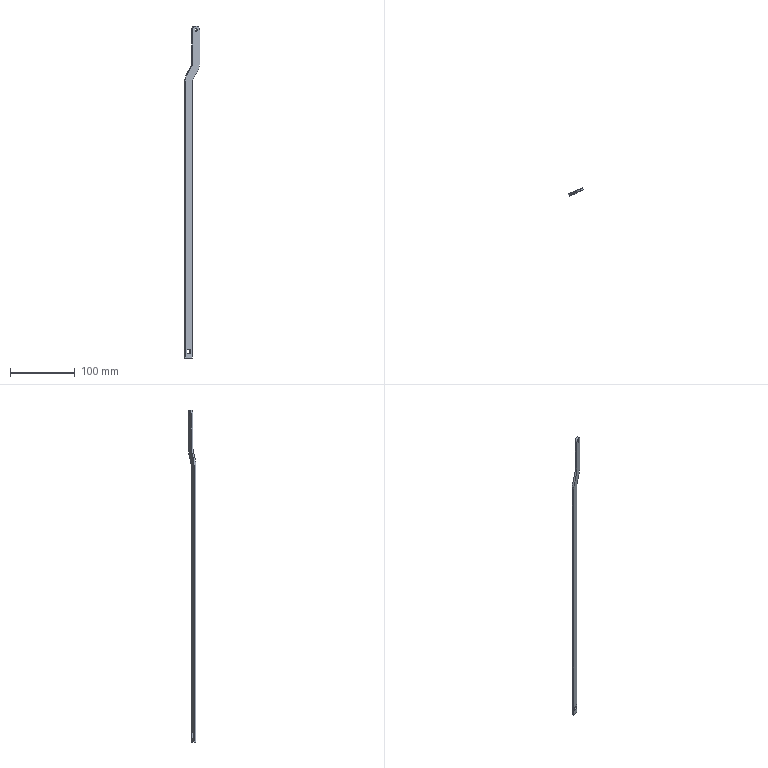Component | SolidWorks | RightDoorAssembly-1_LinkRodLock-1_UpperLinkRod-1 | 1 solid | 21 faces | box 23.38 x 11.77 x 511 mm | volume 18287 mm3 | plane 13 | cylinder 8 | commonest cylinder face diameters 4.2 x2 12 x2 10 x2 34 x2
STEP:
#1=COLOUR_RGB('',0.7922,0.8196,0.9333);
#2=FILL_AREA_STYLE_COLOUR('',#1);
#3=FILL_AREA_STYLE('',(#2));
#4=SURFACE_STYLE_FILL_AREA(#3);
#5=SURFACE_SIDE_STYLE('',(#4));
#6=SURFACE_STYLE_USAGE(.BOTH.,#5);
#7=PRESENTATION_STYLE_ASSIGNMENT((#6));
#8=CARTESIAN_POINT('',(-12.373,15.98,59.984));
#9=VERTEX_POINT('',#8);
#10=CARTESIAN_POINT('',(-12.373,15.98,60.15));
#11=VERTEX_POINT('',#10);
#12=CARTESIAN_POINT('',(-12.373,15.98,60.067));
#13=DIRECTION('',(-0.3744,0.9273,-0.));
#14=DIRECTION('',(0.,0.,1.));
#15=AXIS2_PLACEMENT_3D('',#12,#13,#14);
#16=CIRCLE('',#15,0.08268);
#17=EDGE_CURVE('',#9,#11,#16,.T.);
#18=ORIENTED_EDGE('',*,*,#17,.F.);
#19=CARTESIAN_POINT('',(-12.417,16.09,59.984));
#20=VERTEX_POINT('',#19);
#21=CARTESIAN_POINT('',(-12.373,15.98,59.984));
#22=DIRECTION('',(-0.3744,0.9273,-0.));
#23=VECTOR('',#22,39.37);
#24=LINE('',#21,#23);
#25=EDGE_CURVE('',#9,#20,#24,.T.);
#26=ORIENTED_EDGE('',*,*,#25,.T.);
#27=CARTESIAN_POINT('',(-12.417,16.09,60.15));
#28=VERTEX_POINT('',#27);
#29=CARTESIAN_POINT('',(-12.417,16.09,60.067));
#30=DIRECTION('',(-0.3744,0.9273,-0.));
#31=DIRECTION('',(0.,0.,1.));
#32=AXIS2_PLACEMENT_3D('',#29,#30,#31);
#33=CIRCLE('',#32,0.08268);
#34=EDGE_CURVE('',#20,#28,#33,.T.);
#35=ORIENTED_EDGE('',*,*,#34,.T.);
#36=CARTESIAN_POINT('',(-12.373,15.98,60.15));
#37=DIRECTION('',(-0.3744,0.9273,-0.));
#38=VECTOR('',#37,39.37);
#39=LINE('',#36,#38);
#40=EDGE_CURVE('',#11,#28,#39,.T.);
#41=ORIENTED_EDGE('',*,*,#40,.F.);
#42=EDGE_LOOP('',(#18,#26,#35,#41));
#43=FACE_OUTER_BOUND('',#42,.T.);
#44=CARTESIAN_POINT('',(-12.373,15.98,60.067));
#45=DIRECTION('',(-0.3744,0.9273,-0.));
#46=DIRECTION('',(0.,0.,1.));
#47=AXIS2_PLACEMENT_3D('',#44,#45,#46);
#48=CYLINDRICAL_SURFACE('',#47,0.08268);
#49=ADVANCED_FACE('',(#43),#48,.F.);
#50=CARTESIAN_POINT('',(-12.592,15.892,60.067));
#51=VERTEX_POINT('',#50);
#52=CARTESIAN_POINT('',(-12.373,15.98,60.303));
#53=VERTEX_POINT('',#52);
#54=CARTESIAN_POINT('',(-12.373,15.98,60.067));
#55=DIRECTION('',(-0.3744,0.9273,-0.));
#56=DIRECTION('',(-0.,0.,1.));
#57=AXIS2_PLACEMENT_3D('',#54,#55,#56);
#58=CIRCLE('',#57,0.2362);
#59=EDGE_CURVE('',#51,#53,#58,.T.);
#60=ORIENTED_EDGE('',*,*,#59,.T.);
#61=CARTESIAN_POINT('',(-12.417,16.09,60.303));
#62=VERTEX_POINT('',#61);
#63=CARTESIAN_POINT('',(-12.373,15.98,60.303));
#64=DIRECTION('',(-0.3744,0.9273,-0.));
#65=VECTOR('',#64,39.37);
#66=LINE('',#63,#65);
#67=EDGE_CURVE('',#53,#62,#66,.T.);
#68=ORIENTED_EDGE('',*,*,#67,.T.);
#69=CARTESIAN_POINT('',(-12.636,16.001,60.067));
#70=VERTEX_POINT('',#69);
#71=CARTESIAN_POINT('',(-12.417,16.09,60.067));
#72=DIRECTION('',(-0.3744,0.9273,-0.));
#73=DIRECTION('',(-0.,0.,1.));
#74=AXIS2_PLACEMENT_3D('',#71,#72,#73);
#75=CIRCLE('',#74,0.2362);
#76=EDGE_CURVE('',#70,#62,#75,.T.);
#77=ORIENTED_EDGE('',*,*,#76,.F.);
#78=CARTESIAN_POINT('',(-12.592,15.892,60.067));
#79=DIRECTION('',(-0.3744,0.9273,-0.));
#80=VECTOR('',#79,39.37);
#81=LINE('',#78,#80);
#82=EDGE_CURVE('',#51,#70,#81,.T.);
#83=ORIENTED_EDGE('',*,*,#82,.F.);
#84=EDGE_LOOP('',(#60,#68,#77,#83));
#85=FACE_OUTER_BOUND('',#84,.T.);
#86=CARTESIAN_POINT('',(-12.373,15.98,60.067));
#87=DIRECTION('',(-0.3744,0.9273,-0.));
#88=DIRECTION('',(-0.,0.,1.));
#89=AXIS2_PLACEMENT_3D('',#86,#87,#88);
#90=CYLINDRICAL_SURFACE('',#89,0.2362);
#91=ADVANCED_FACE('',(#85),#90,.T.);
#92=CARTESIAN_POINT('',(-13.074,15.824,40.185));
#93=VERTEX_POINT('',#92);
#94=CARTESIAN_POINT('',(-13.074,15.824,56.942));
#95=VERTEX_POINT('',#94);
#96=CARTESIAN_POINT('',(-13.074,15.824,40.185));
#97=DIRECTION('',(-0.,0.,1.));
#98=VECTOR('',#97,39.37);
#99=LINE('',#96,#98);
#100=EDGE_CURVE('',#93,#95,#99,.T.);
#101=ORIENTED_EDGE('',*,*,#100,.F.);
#102=CARTESIAN_POINT('',(-13.03,15.715,40.185));
#103=VERTEX_POINT('',#102);
#104=CARTESIAN_POINT('',(-13.03,15.715,40.185));
#105=DIRECTION('',(-0.3744,0.9273,-0.));
#106=VECTOR('',#105,39.37);
#107=LINE('',#104,#106);
#108=EDGE_CURVE('',#103,#93,#107,.T.);
#109=ORIENTED_EDGE('',*,*,#108,.F.);
#110=CARTESIAN_POINT('',(-13.03,15.715,56.942));
#111=VERTEX_POINT('',#110);
#112=CARTESIAN_POINT('',(-13.03,15.715,40.185));
#113=DIRECTION('',(-0.,0.,1.));
#114=VECTOR('',#113,39.37);
#115=LINE('',#112,#114);
#116=EDGE_CURVE('',#103,#111,#115,.T.);
#117=ORIENTED_EDGE('',*,*,#116,.T.);
#118=CARTESIAN_POINT('',(-13.03,15.715,56.942));
#119=DIRECTION('',(-0.3744,0.9273,-0.));
#120=VECTOR('',#119,39.37);
#121=LINE('',#118,#120);
#122=EDGE_CURVE('',#111,#95,#121,.T.);
#123=ORIENTED_EDGE('',*,*,#122,.T.);
#124=EDGE_LOOP('',(#101,#109,#117,#123));
#125=FACE_OUTER_BOUND('',#124,.T.);
#126=CARTESIAN_POINT('',(-13.03,15.715,40.185));
#127=DIRECTION('',(-0.9273,-0.3744,-0.));
#128=DIRECTION('',(-0.,0.,1.));
#129=AXIS2_PLACEMENT_3D('',#126,#127,#128);
#130=PLANE('',#129);
#131=ADVANCED_FACE('',(#125),#130,.T.);
#132=CARTESIAN_POINT('',(-12.636,16.001,40.185));
#133=VERTEX_POINT('',#132);
#134=CARTESIAN_POINT('',(-12.636,16.001,40.185));
#135=DIRECTION('',(-0.9273,-0.3744,-0.));
#136=VECTOR('',#135,39.37);
#137=LINE('',#134,#136);
#138=EDGE_CURVE('',#133,#93,#137,.T.);
#139=ORIENTED_EDGE('',*,*,#138,.F.);
#140=CARTESIAN_POINT('',(-12.592,15.892,40.185));
#141=VERTEX_POINT('',#140);
#142=CARTESIAN_POINT('',(-12.592,15.892,40.185));
#143=DIRECTION('',(-0.3744,0.9273,-0.));
#144=VECTOR('',#143,39.37);
#145=LINE('',#142,#144);
#146=EDGE_CURVE('',#141,#133,#145,.T.);
#147=ORIENTED_EDGE('',*,*,#146,.F.);
#148=CARTESIAN_POINT('',(-12.592,15.892,40.185));
#149=DIRECTION('',(-0.9273,-0.3744,-0.));
#150=VECTOR('',#149,39.37);
#151=LINE('',#148,#150);
#152=EDGE_CURVE('',#141,#103,#151,.T.);
#153=ORIENTED_EDGE('',*,*,#152,.T.);
#154=ORIENTED_EDGE('',*,*,#108,.T.);
#155=EDGE_LOOP('',(#139,#147,#153,#154));
#156=FACE_OUTER_BOUND('',#155,.T.);
#157=CARTESIAN_POINT('',(-12.592,15.892,40.185));
#158=DIRECTION('',(0.,-0.,-1.));
#159=DIRECTION('',(-0.3744,0.9273,-0.));
#160=AXIS2_PLACEMENT_3D('',#157,#158,#159);
#161=PLANE('',#160);
#162=ADVANCED_FACE('',(#156),#161,.T.);
#163=CARTESIAN_POINT('',(-12.636,16.001,56.942));
#164=VERTEX_POINT('',#163);
#165=CARTESIAN_POINT('',(-12.636,16.001,40.185));
#166=DIRECTION('',(0.,-0.,-1.));
#167=VECTOR('',#166,39.37);
#168=LINE('',#165,#167);
#169=EDGE_CURVE('',#164,#133,#168,.T.);
#170=ORIENTED_EDGE('',*,*,#169,.F.);
#171=CARTESIAN_POINT('',(-12.592,15.892,56.942));
#172=VERTEX_POINT('',#171);
#173=CARTESIAN_POINT('',(-12.592,15.892,56.942));
#174=DIRECTION('',(-0.3744,0.9273,-0.));
#175=VECTOR('',#174,39.37);
#176=LINE('',#173,#175);
#177=EDGE_CURVE('',#172,#164,#176,.T.);
#178=ORIENTED_EDGE('',*,*,#177,.F.);
#179=CARTESIAN_POINT('',(-12.592,15.892,40.185));
#180=DIRECTION('',(0.,-0.,-1.));
#181=VECTOR('',#180,39.37);
#182=LINE('',#179,#181);
#183=EDGE_CURVE('',#172,#141,#182,.T.);
#184=ORIENTED_EDGE('',*,*,#183,.T.);
#185=ORIENTED_EDGE('',*,*,#146,.T.);
#186=EDGE_LOOP('',(#170,#178,#184,#185));
#187=FACE_OUTER_BOUND('',#186,.T.);
#188=CARTESIAN_POINT('',(-12.592,15.892,40.185));
#189=DIRECTION('',(0.9273,0.3744,0.));
#190=DIRECTION('',(0.,-0.,-1.));
#191=AXIS2_PLACEMENT_3D('',#188,#189,#190);
#192=PLANE('',#191);
#193=ADVANCED_FACE('',(#187),#192,.T.);
#194=CARTESIAN_POINT('',(-12.612,16.011,57.04));
#195=VERTEX_POINT('',#194);
#196=CARTESIAN_POINT('',(-12.454,16.075,56.942));
#197=DIRECTION('',(0.3744,-0.9273,0.));
#198=DIRECTION('',(-0.,0.,1.));
#199=AXIS2_PLACEMENT_3D('',#196,#197,#198);
#200=CIRCLE('',#199,0.1969);
#201=EDGE_CURVE('',#195,#164,#200,.T.);
#202=ORIENTED_EDGE('',*,*,#201,.F.);
#203=CARTESIAN_POINT('',(-12.568,15.902,57.04));
#204=VERTEX_POINT('',#203);
#205=CARTESIAN_POINT('',(-12.568,15.902,57.04));
#206=DIRECTION('',(-0.3744,0.9273,-0.));
#207=VECTOR('',#206,39.37);
#208=LINE('',#205,#207);
#209=EDGE_CURVE('',#204,#195,#208,.T.);
#210=ORIENTED_EDGE('',*,*,#209,.F.);
#211=CARTESIAN_POINT('',(-12.41,15.965,56.942));
#212=DIRECTION('',(0.3744,-0.9273,0.));
#213=DIRECTION('',(-0.,0.,1.));
#214=AXIS2_PLACEMENT_3D('',#211,#212,#213);
#215=CIRCLE('',#214,0.1969);
#216=EDGE_CURVE('',#204,#172,#215,.T.);
#217=ORIENTED_EDGE('',*,*,#216,.T.);
#218=ORIENTED_EDGE('',*,*,#177,.T.);
#219=EDGE_LOOP('',(#202,#210,#217,#218));
#220=FACE_OUTER_BOUND('',#219,.T.);
#221=CARTESIAN_POINT('',(-12.41,15.965,56.942));
#222=DIRECTION('',(-0.3744,0.9273,-0.));
#223=DIRECTION('',(-0.,0.,1.));
#224=AXIS2_PLACEMENT_3D('',#221,#222,#223);
#225=CYLINDRICAL_SURFACE('',#224,0.1969);
#226=ADVANCED_FACE('',(#220),#225,.F.);
#227=CARTESIAN_POINT('',(-12.281,16.145,57.657));
#228=VERTEX_POINT('',#227);
#229=CARTESIAN_POINT('',(-12.281,16.145,57.657));
#230=DIRECTION('',(-0.4636,-0.1872,-0.866));
#231=VECTOR('',#230,39.37);
#232=LINE('',#229,#231);
#233=EDGE_CURVE('',#228,#195,#232,.T.);
#234=ORIENTED_EDGE('',*,*,#233,.F.);
#235=CARTESIAN_POINT('',(-12.237,16.035,57.657));
#236=VERTEX_POINT('',#235);
#237=CARTESIAN_POINT('',(-12.237,16.035,57.657));
#238=DIRECTION('',(-0.3744,0.9273,-0.));
#239=VECTOR('',#238,39.37);
#240=LINE('',#237,#239);
#241=EDGE_CURVE('',#236,#228,#240,.T.);
#242=ORIENTED_EDGE('',*,*,#241,.F.);
#243=CARTESIAN_POINT('',(-12.237,16.035,57.657));
#244=DIRECTION('',(-0.4636,-0.1872,-0.866));
#245=VECTOR('',#244,39.37);
#246=LINE('',#243,#245);
#247=EDGE_CURVE('',#236,#204,#246,.T.);
#248=ORIENTED_EDGE('',*,*,#247,.T.);
#249=ORIENTED_EDGE('',*,*,#209,.T.);
#250=EDGE_LOOP('',(#234,#242,#248,#249));
#251=FACE_OUTER_BOUND('',#250,.T.);
#252=CARTESIAN_POINT('',(-12.237,16.035,57.657));
#253=DIRECTION('',(0.803,0.3242,-0.5));
#254=DIRECTION('',(-0.4636,-0.1872,-0.866));
#255=AXIS2_PLACEMENT_3D('',#252,#253,#254);
#256=PLANE('',#255);
#257=ADVANCED_FACE('',(#251),#256,.T.);
#258=CARTESIAN_POINT('',(-12.198,16.178,57.992));
#259=VERTEX_POINT('',#258);
#260=CARTESIAN_POINT('',(-12.819,15.928,57.992));
#261=DIRECTION('',(-0.3744,0.9273,-0.));
#262=DIRECTION('',(-0.,0.,1.));
#263=AXIS2_PLACEMENT_3D('',#260,#261,#262);
#264=CIRCLE('',#263,0.6693);
#265=EDGE_CURVE('',#259,#228,#264,.T.);
#266=ORIENTED_EDGE('',*,*,#265,.F.);
#267=CARTESIAN_POINT('',(-12.154,16.069,57.992));
#268=VERTEX_POINT('',#267);
#269=CARTESIAN_POINT('',(-12.154,16.069,57.992));
#270=DIRECTION('',(-0.3744,0.9273,-0.));
#271=VECTOR('',#270,39.37);
#272=LINE('',#269,#271);
#273=EDGE_CURVE('',#268,#259,#272,.T.);
#274=ORIENTED_EDGE('',*,*,#273,.F.);
#275=CARTESIAN_POINT('',(-12.775,15.818,57.992));
#276=DIRECTION('',(-0.3744,0.9273,-0.));
#277=DIRECTION('',(-0.,0.,1.));
#278=AXIS2_PLACEMENT_3D('',#275,#276,#277);
#279=CIRCLE('',#278,0.6693);
#280=EDGE_CURVE('',#268,#236,#279,.T.);
#281=ORIENTED_EDGE('',*,*,#280,.T.);
#282=ORIENTED_EDGE('',*,*,#241,.T.);
#283=EDGE_LOOP('',(#266,#274,#281,#282));
#284=FACE_OUTER_BOUND('',#283,.T.);
#285=CARTESIAN_POINT('',(-12.775,15.818,57.992));
#286=DIRECTION('',(-0.3744,0.9273,-0.));
#287=DIRECTION('',(-0.,0.,1.));
#288=AXIS2_PLACEMENT_3D('',#285,#286,#287);
#289=CYLINDRICAL_SURFACE('',#288,0.6693);
#290=ADVANCED_FACE('',(#284),#289,.T.);
#291=CARTESIAN_POINT('',(-12.198,16.178,60.067));
#292=VERTEX_POINT('',#291);
#293=CARTESIAN_POINT('',(-12.198,16.178,57.992));
#294=DIRECTION('',(0.,-0.,-1.));
#295=VECTOR('',#294,39.37);
#296=LINE('',#293,#295);
#297=EDGE_CURVE('',#292,#259,#296,.T.);
#298=ORIENTED_EDGE('',*,*,#297,.F.);
#299=CARTESIAN_POINT('',(-12.154,16.069,60.067));
#300=VERTEX_POINT('',#299);
#301=CARTESIAN_POINT('',(-12.154,16.069,60.067));
#302=DIRECTION('',(-0.3744,0.9273,-0.));
#303=VECTOR('',#302,39.37);
#304=LINE('',#301,#303);
#305=EDGE_CURVE('',#300,#292,#304,.T.);
#306=ORIENTED_EDGE('',*,*,#305,.F.);
#307=CARTESIAN_POINT('',(-12.154,16.069,57.992));
#308=DIRECTION('',(0.,-0.,-1.));
#309=VECTOR('',#308,39.37);
#310=LINE('',#307,#309);
#311=EDGE_CURVE('',#300,#268,#310,.T.);
#312=ORIENTED_EDGE('',*,*,#311,.T.);
#313=ORIENTED_EDGE('',*,*,#273,.T.);
#314=EDGE_LOOP('',(#298,#306,#312,#313));
#315=FACE_OUTER_BOUND('',#314,.T.);
#316=CARTESIAN_POINT('',(-12.154,16.069,57.992));
#317=DIRECTION('',(0.9273,0.3744,0.));
#318=DIRECTION('',(0.,-0.,-1.));
#319=AXIS2_PLACEMENT_3D('',#316,#317,#318);
#320=PLANE('',#319);
#321=ADVANCED_FACE('',(#315),#320,.T.);
#322=ORIENTED_EDGE('',*,*,#67,.F.);
#323=CARTESIAN_POINT('',(-12.373,15.98,60.067));
#324=DIRECTION('',(-0.3744,0.9273,-0.));
#325=DIRECTION('',(-0.,0.,1.));
#326=AXIS2_PLACEMENT_3D('',#323,#324,#325);
#327=CIRCLE('',#326,0.2362);
#328=EDGE_CURVE('',#53,#300,#327,.T.);
#329=ORIENTED_EDGE('',*,*,#328,.T.);
#330=ORIENTED_EDGE('',*,*,#305,.T.);
#331=CARTESIAN_POINT('',(-12.417,16.09,60.067));
#332=DIRECTION('',(-0.3744,0.9273,-0.));
#333=DIRECTION('',(-0.,0.,1.));
#334=AXIS2_PLACEMENT_3D('',#331,#332,#333);
#335=CIRCLE('',#334,0.2362);
#336=EDGE_CURVE('',#62,#292,#335,.T.);
#337=ORIENTED_EDGE('',*,*,#336,.F.);
#338=EDGE_LOOP('',(#322,#329,#330,#337));
#339=FACE_OUTER_BOUND('',#338,.T.);
#340=CARTESIAN_POINT('',(-12.373,15.98,60.067));
#341=DIRECTION('',(-0.3744,0.9273,-0.));
#342=DIRECTION('',(-0.,0.,1.));
#343=AXIS2_PLACEMENT_3D('',#340,#341,#342);
#344=CYLINDRICAL_SURFACE('',#343,0.2362);
#345=ADVANCED_FACE('',(#339),#344,.T.);
#346=CARTESIAN_POINT('',(-12.636,16.001,57.992));
#347=VERTEX_POINT('',#346);
#348=CARTESIAN_POINT('',(-12.636,16.001,57.992));
#349=DIRECTION('',(0.,0.,1.));
#350=VECTOR('',#349,39.37);
#351=LINE('',#348,#350);
#352=EDGE_CURVE('',#347,#70,#351,.T.);
#353=ORIENTED_EDGE('',*,*,#352,.F.);
#354=CARTESIAN_POINT('',(-12.592,15.892,57.992));
#355=VERTEX_POINT('',#354);
#356=CARTESIAN_POINT('',(-12.592,15.892,57.992));
#357=DIRECTION('',(-0.3744,0.9273,-0.));
#358=VECTOR('',#357,39.37);
#359=LINE('',#356,#358);
#360=EDGE_CURVE('',#355,#347,#359,.T.);
#361=ORIENTED_EDGE('',*,*,#360,.F.);
#362=CARTESIAN_POINT('',(-12.592,15.892,57.992));
#363=DIRECTION('',(0.,0.,1.));
#364=VECTOR('',#363,39.37);
#365=LINE('',#362,#364);
#366=EDGE_CURVE('',#355,#51,#365,.T.);
#367=ORIENTED_EDGE('',*,*,#366,.T.);
#368=ORIENTED_EDGE('',*,*,#82,.T.);
#369=EDGE_LOOP('',(#353,#361,#367,#368));
#370=FACE_OUTER_BOUND('',#369,.T.);
#371=CARTESIAN_POINT('',(-12.592,15.892,57.992));
#372=DIRECTION('',(-0.9273,-0.3744,0.));
#373=DIRECTION('',(0.,0.,1.));
#374=AXIS2_PLACEMENT_3D('',#371,#372,#373);
#375=PLANE('',#374);
#376=ADVANCED_FACE('',(#370),#375,.T.);
#377=CARTESIAN_POINT('',(-12.661,15.991,57.894));
#378=VERTEX_POINT('',#377);
#379=CARTESIAN_POINT('',(-12.819,15.928,57.992));
#380=DIRECTION('',(0.3744,-0.9273,0.));
#381=DIRECTION('',(-0.,0.,1.));
#382=AXIS2_PLACEMENT_3D('',#379,#380,#381);
#383=CIRCLE('',#382,0.1969);
#384=EDGE_CURVE('',#378,#347,#383,.T.);
#385=ORIENTED_EDGE('',*,*,#384,.F.);
#386=CARTESIAN_POINT('',(-12.617,15.882,57.894));
#387=VERTEX_POINT('',#386);
#388=CARTESIAN_POINT('',(-12.617,15.882,57.894));
#389=DIRECTION('',(-0.3744,0.9273,-0.));
#390=VECTOR('',#389,39.37);
#391=LINE('',#388,#390);
#392=EDGE_CURVE('',#387,#378,#391,.T.);
#393=ORIENTED_EDGE('',*,*,#392,.F.);
#394=CARTESIAN_POINT('',(-12.775,15.818,57.992));
#395=DIRECTION('',(0.3744,-0.9273,0.));
#396=DIRECTION('',(-0.,0.,1.));
#397=AXIS2_PLACEMENT_3D('',#394,#395,#396);
#398=CIRCLE('',#397,0.1969);
#399=EDGE_CURVE('',#387,#355,#398,.T.);
#400=ORIENTED_EDGE('',*,*,#399,.T.);
#401=ORIENTED_EDGE('',*,*,#360,.T.);
#402=EDGE_LOOP('',(#385,#393,#400,#401));
#403=FACE_OUTER_BOUND('',#402,.T.);
#404=CARTESIAN_POINT('',(-12.775,15.818,57.992));
#405=DIRECTION('',(-0.3744,0.9273,-0.));
#406=DIRECTION('',(-0.,0.,1.));
#407=AXIS2_PLACEMENT_3D('',#404,#405,#406);
#408=CYLINDRICAL_SURFACE('',#407,0.1969);
#409=ADVANCED_FACE('',(#403),#408,.F.);
#410=CARTESIAN_POINT('',(-12.991,15.858,57.276));
#411=VERTEX_POINT('',#410);
#412=CARTESIAN_POINT('',(-12.661,15.991,57.894));
#413=DIRECTION('',(0.4636,0.1872,0.866));
#414=VECTOR('',#413,39.37);
#415=LINE('',#412,#414);
#416=EDGE_CURVE('',#411,#378,#415,.T.);
#417=ORIENTED_EDGE('',*,*,#416,.F.);
#418=CARTESIAN_POINT('',(-12.947,15.748,57.276));
#419=VERTEX_POINT('',#418);
#420=CARTESIAN_POINT('',(-12.947,15.748,57.276));
#421=DIRECTION('',(-0.3744,0.9273,-0.));
#422=VECTOR('',#421,39.37);
#423=LINE('',#420,#422);
#424=EDGE_CURVE('',#419,#411,#423,.T.);
#425=ORIENTED_EDGE('',*,*,#424,.F.);
#426=CARTESIAN_POINT('',(-12.617,15.882,57.894));
#427=DIRECTION('',(0.4636,0.1872,0.866));
#428=VECTOR('',#427,39.37);
#429=LINE('',#426,#428);
#430=EDGE_CURVE('',#419,#387,#429,.T.);
#431=ORIENTED_EDGE('',*,*,#430,.T.);
#432=ORIENTED_EDGE('',*,*,#392,.T.);
#433=EDGE_LOOP('',(#417,#425,#431,#432));
#434=FACE_OUTER_BOUND('',#433,.T.);
#435=CARTESIAN_POINT('',(-12.617,15.882,57.894));
#436=DIRECTION('',(-0.803,-0.3242,0.5));
#437=DIRECTION('',(0.4636,0.1872,0.866));
#438=AXIS2_PLACEMENT_3D('',#435,#436,#437);
#439=PLANE('',#438);
#440=ADVANCED_FACE('',(#434),#439,.T.);
#441=CARTESIAN_POINT('',(-12.454,16.075,56.942));
#442=DIRECTION('',(-0.3744,0.9273,-0.));
#443=DIRECTION('',(-0.,0.,1.));
#444=AXIS2_PLACEMENT_3D('',#441,#442,#443);
#445=CIRCLE('',#444,0.6693);
#446=EDGE_CURVE('',#95,#411,#445,.T.);
#447=ORIENTED_EDGE('',*,*,#446,.F.);
#448=ORIENTED_EDGE('',*,*,#122,.F.);
#449=CARTESIAN_POINT('',(-12.41,15.965,56.942));
#450=DIRECTION('',(-0.3744,0.9273,-0.));
#451=DIRECTION('',(-0.,0.,1.));
#452=AXIS2_PLACEMENT_3D('',#449,#450,#451);
#453=CIRCLE('',#452,0.6693);
#454=EDGE_CURVE('',#111,#419,#453,.T.);
#455=ORIENTED_EDGE('',*,*,#454,.T.);
#456=ORIENTED_EDGE('',*,*,#424,.T.);
#457=EDGE_LOOP('',(#447,#448,#455,#456));
#458=FACE_OUTER_BOUND('',#457,.T.);
#459=CARTESIAN_POINT('',(-12.41,15.965,56.942));
#460=DIRECTION('',(-0.3744,0.9273,-0.));
#461=DIRECTION('',(-0.,0.,1.));
#462=AXIS2_PLACEMENT_3D('',#459,#460,#461);
#463=CYLINDRICAL_SURFACE('',#462,0.6693);
#464=ADVANCED_FACE('',(#458),#463,.T.);
#465=CARTESIAN_POINT('',(-12.373,15.98,60.067));
#466=DIRECTION('',(-0.3744,0.9273,-0.));
#467=DIRECTION('',(0.,0.,1.));
#468=AXIS2_PLACEMENT_3D('',#465,#466,#467);
#469=CIRCLE('',#468,0.08268);
#470=EDGE_CURVE('',#11,#9,#469,.T.);
#471=ORIENTED_EDGE('',*,*,#470,.T.);
#472=ORIENTED_EDGE('',*,*,#17,.T.);
#473=EDGE_LOOP('',(#471,#472));
#474=FACE_BOUND('',#473,.T.);
#475=CARTESIAN_POINT('',(-12.93,15.755,40.707));
#476=VERTEX_POINT('',#475);
#477=CARTESIAN_POINT('',(-12.693,15.851,40.707));
#478=VERTEX_POINT('',#477);
#479=CARTESIAN_POINT('',(-12.693,15.851,40.707));
#480=DIRECTION('',(0.9273,0.3744,0.));
#481=VECTOR('',#480,39.37);
#482=LINE('',#479,#481);
#483=EDGE_CURVE('',#476,#478,#482,.T.);
#484=ORIENTED_EDGE('',*,*,#483,.T.);
#485=CARTESIAN_POINT('',(-12.693,15.851,40.451));
#486=VERTEX_POINT('',#485);
#487=CARTESIAN_POINT('',(-12.693,15.851,40.451));
#488=DIRECTION('',(0.,-0.,-1.));
#489=VECTOR('',#488,39.37);
#490=LINE('',#487,#489);
#491=EDGE_CURVE('',#478,#486,#490,.T.);
#492=ORIENTED_EDGE('',*,*,#491,.T.);
#493=CARTESIAN_POINT('',(-12.93,15.755,40.451));
#494=VERTEX_POINT('',#493);
#495=CARTESIAN_POINT('',(-12.93,15.755,40.451));
#496=DIRECTION('',(-0.9273,-0.3744,-0.));
#497=VECTOR('',#496,39.37);
#498=LINE('',#495,#497);
#499=EDGE_CURVE('',#486,#494,#498,.T.);
#500=ORIENTED_EDGE('',*,*,#499,.T.);
#501=CARTESIAN_POINT('',(-12.93,15.755,40.707));
#502=DIRECTION('',(-0.,0.,1.));
#503=VECTOR('',#502,39.37);
#504=LINE('',#501,#503);
#505=EDGE_CURVE('',#494,#476,#504,.T.);
#506=ORIENTED_EDGE('',*,*,#505,.T.);
#507=EDGE_LOOP('',(#484,#492,#500,#506));
#508=FACE_BOUND('',#507,.T.);
#509=ORIENTED_EDGE('',*,*,#116,.F.);
#510=ORIENTED_EDGE('',*,*,#152,.F.);
#511=ORIENTED_EDGE('',*,*,#183,.F.);
#512=ORIENTED_EDGE('',*,*,#216,.F.);
#513=ORIENTED_EDGE('',*,*,#247,.F.);
#514=ORIENTED_EDGE('',*,*,#280,.F.);
#515=ORIENTED_EDGE('',*,*,#311,.F.);
#516=ORIENTED_EDGE('',*,*,#328,.F.);
#517=ORIENTED_EDGE('',*,*,#59,.F.);
#518=ORIENTED_EDGE('',*,*,#366,.F.);
#519=ORIENTED_EDGE('',*,*,#399,.F.);
#520=ORIENTED_EDGE('',*,*,#430,.F.);
#521=ORIENTED_EDGE('',*,*,#454,.F.);
#522=EDGE_LOOP('',(#509,#510,#511,#512,#513,#514,#515,#516,#517,#518,#519,#520,#521));
#523=FACE_OUTER_BOUND('',#522,.T.);
#524=CARTESIAN_POINT('',(-12.41,15.965,56.942));
#525=DIRECTION('',(-0.3744,0.9273,-0.));
#526=DIRECTION('',(-0.,0.,1.));
#527=AXIS2_PLACEMENT_3D('',#524,#525,#526);
#528=PLANE('',#527);
#529=ADVANCED_FACE('',(#474,#508,#523),#528,.F.);
#530=CARTESIAN_POINT('',(-12.417,16.09,60.067));
#531=DIRECTION('',(-0.3744,0.9273,-0.));
#532=DIRECTION('',(0.,0.,1.));
#533=AXIS2_PLACEMENT_3D('',#530,#531,#532);
#534=CIRCLE('',#533,0.08268);
#535=EDGE_CURVE('',#28,#20,#534,.T.);
#536=ORIENTED_EDGE('',*,*,#535,.F.);
#537=ORIENTED_EDGE('',*,*,#34,.F.);
#538=EDGE_LOOP('',(#536,#537));
#539=FACE_BOUND('',#538,.T.);
#540=CARTESIAN_POINT('',(-12.737,15.961,40.707));
#541=VERTEX_POINT('',#540);
#542=CARTESIAN_POINT('',(-12.737,15.961,40.451));
#543=VERTEX_POINT('',#542);
#544=CARTESIAN_POINT('',(-12.737,15.961,40.451));
#545=DIRECTION('',(0.,-0.,-1.));
#546=VECTOR('',#545,39.37);
#547=LINE('',#544,#546);
#548=EDGE_CURVE('',#541,#543,#547,.T.);
#549=ORIENTED_EDGE('',*,*,#548,.F.);
#550=CARTESIAN_POINT('',(-12.974,15.865,40.707));
#551=VERTEX_POINT('',#550);
#552=CARTESIAN_POINT('',(-12.737,15.961,40.707));
#553=DIRECTION('',(0.9273,0.3744,0.));
#554=VECTOR('',#553,39.37);
#555=LINE('',#552,#554);
#556=EDGE_CURVE('',#551,#541,#555,.T.);
#557=ORIENTED_EDGE('',*,*,#556,.F.);
#558=CARTESIAN_POINT('',(-12.974,15.865,40.451));
#559=VERTEX_POINT('',#558);
#560=CARTESIAN_POINT('',(-12.974,15.865,40.707));
#561=DIRECTION('',(-0.,0.,1.));
#562=VECTOR('',#561,39.37);
#563=LINE('',#560,#562);
#564=EDGE_CURVE('',#559,#551,#563,.T.);
#565=ORIENTED_EDGE('',*,*,#564,.F.);
#566=CARTESIAN_POINT('',(-12.974,15.865,40.451));
#567=DIRECTION('',(-0.9273,-0.3744,-0.));
#568=VECTOR('',#567,39.37);
#569=LINE('',#566,#568);
#570=EDGE_CURVE('',#543,#559,#569,.T.);
#571=ORIENTED_EDGE('',*,*,#570,.F.);
#572=EDGE_LOOP('',(#549,#557,#565,#571));
#573=FACE_BOUND('',#572,.T.);
#574=ORIENTED_EDGE('',*,*,#100,.T.);
#575=ORIENTED_EDGE('',*,*,#446,.T.);
#576=ORIENTED_EDGE('',*,*,#416,.T.);
#577=ORIENTED_EDGE('',*,*,#384,.T.);
#578=ORIENTED_EDGE('',*,*,#352,.T.);
#579=ORIENTED_EDGE('',*,*,#76,.T.);
#580=ORIENTED_EDGE('',*,*,#336,.T.);
#581=ORIENTED_EDGE('',*,*,#297,.T.);
#582=ORIENTED_EDGE('',*,*,#265,.T.);
#583=ORIENTED_EDGE('',*,*,#233,.T.);
#584=ORIENTED_EDGE('',*,*,#201,.T.);
#585=ORIENTED_EDGE('',*,*,#169,.T.);
#586=ORIENTED_EDGE('',*,*,#138,.T.);
#587=EDGE_LOOP('',(#574,#575,#576,#577,#578,#579,#580,#581,#582,#583,#584,#585,#586));
#588=FACE_OUTER_BOUND('',#587,.T.);
#589=CARTESIAN_POINT('',(-12.454,16.075,56.942));
#590=DIRECTION('',(-0.3744,0.9273,-0.));
#591=DIRECTION('',(-0.,0.,1.));
#592=AXIS2_PLACEMENT_3D('',#589,#590,#591);
#593=PLANE('',#592);
#594=ADVANCED_FACE('',(#539,#573,#588),#593,.T.);
#595=ORIENTED_EDGE('',*,*,#548,.T.);
#596=CARTESIAN_POINT('',(-12.693,15.851,40.451));
#597=DIRECTION('',(-0.3744,0.9273,-0.));
#598=VECTOR('',#597,39.37);
#599=LINE('',#596,#598);
#600=EDGE_CURVE('',#486,#543,#599,.T.);
#601=ORIENTED_EDGE('',*,*,#600,.F.);
#602=ORIENTED_EDGE('',*,*,#491,.F.);
#603=CARTESIAN_POINT('',(-12.693,15.851,40.707));
#604=DIRECTION('',(-0.3744,0.9273,-0.));
#605=VECTOR('',#604,39.37);
#606=LINE('',#603,#605);
#607=EDGE_CURVE('',#478,#541,#606,.T.);
#608=ORIENTED_EDGE('',*,*,#607,.T.);
#609=EDGE_LOOP('',(#595,#601,#602,#608));
#610=FACE_OUTER_BOUND('',#609,.T.);
#611=CARTESIAN_POINT('',(-12.693,15.851,40.451));
#612=DIRECTION('',(0.9273,0.3744,0.));
#613=DIRECTION('',(-0.3744,0.9273,-0.));
#614=AXIS2_PLACEMENT_3D('',#611,#612,#613);
#615=PLANE('',#614);
#616=ADVANCED_FACE('',(#610),#615,.F.);
#617=ORIENTED_EDGE('',*,*,#556,.T.);
#618=ORIENTED_EDGE('',*,*,#607,.F.);
#619=ORIENTED_EDGE('',*,*,#483,.F.);
#620=CARTESIAN_POINT('',(-12.93,15.755,40.707));
#621=DIRECTION('',(-0.3744,0.9273,-0.));
#622=VECTOR('',#621,39.37);
#623=LINE('',#620,#622);
#624=EDGE_CURVE('',#476,#551,#623,.T.);
#625=ORIENTED_EDGE('',*,*,#624,.T.);
#626=EDGE_LOOP('',(#617,#618,#619,#625));
#627=FACE_OUTER_BOUND('',#626,.T.);
#628=CARTESIAN_POINT('',(-12.693,15.851,40.707));
#629=DIRECTION('',(-0.,0.,1.));
#630=DIRECTION('',(0.3744,-0.9273,0.));
#631=AXIS2_PLACEMENT_3D('',#628,#629,#630);
#632=PLANE('',#631);
#633=ADVANCED_FACE('',(#627),#632,.F.);
#634=ORIENTED_EDGE('',*,*,#564,.T.);
#635=ORIENTED_EDGE('',*,*,#624,.F.);
#636=ORIENTED_EDGE('',*,*,#505,.F.);
#637=CARTESIAN_POINT('',(-12.93,15.755,40.451));
#638=DIRECTION('',(-0.3744,0.9273,-0.));
#639=VECTOR('',#638,39.37);
#640=LINE('',#637,#639);
#641=EDGE_CURVE('',#494,#559,#640,.T.);
#642=ORIENTED_EDGE('',*,*,#641,.T.);
#643=EDGE_LOOP('',(#634,#635,#636,#642));
#644=FACE_OUTER_BOUND('',#643,.T.);
#645=CARTESIAN_POINT('',(-12.93,15.755,40.707));
#646=DIRECTION('',(-0.9273,-0.3744,-0.));
#647=DIRECTION('',(-0.,0.,1.));
#648=AXIS2_PLACEMENT_3D('',#645,#646,#647);
#649=PLANE('',#648);
#650=ADVANCED_FACE('',(#644),#649,.F.);
#651=ORIENTED_EDGE('',*,*,#570,.T.);
#652=ORIENTED_EDGE('',*,*,#641,.F.);
#653=ORIENTED_EDGE('',*,*,#499,.F.);
#654=ORIENTED_EDGE('',*,*,#600,.T.);
#655=EDGE_LOOP('',(#651,#652,#653,#654));
#656=FACE_OUTER_BOUND('',#655,.T.);
#657=CARTESIAN_POINT('',(-12.93,15.755,40.451));
#658=DIRECTION('',(0.,-0.,-1.));
#659=DIRECTION('',(-0.3744,0.9273,-0.));
#660=AXIS2_PLACEMENT_3D('',#657,#658,#659);
#661=PLANE('',#660);
#662=ADVANCED_FACE('',(#656),#661,.F.);
#663=ORIENTED_EDGE('',*,*,#25,.F.);
#664=ORIENTED_EDGE('',*,*,#470,.F.);
#665=ORIENTED_EDGE('',*,*,#40,.T.);
#666=ORIENTED_EDGE('',*,*,#535,.T.);
#667=EDGE_LOOP('',(#663,#664,#665,#666));
#668=FACE_OUTER_BOUND('',#667,.T.);
#669=CARTESIAN_POINT('',(-12.373,15.98,60.067));
#670=DIRECTION('',(-0.3744,0.9273,-0.));
#671=DIRECTION('',(0.,0.,1.));
#672=AXIS2_PLACEMENT_3D('',#669,#670,#671);
#673=CYLINDRICAL_SURFACE('',#672,0.08268);
#674=ADVANCED_FACE('',(#668),#673,.F.);
#675=CLOSED_SHELL('',(#49,#91,#131,#162,#193,#226,#257,#290,#321,#345,#376,#409,#440,#464,#529,#594,#616,#633,#650,#662,#674));
#676=MANIFOLD_SOLID_BREP('',#675);
#677=STYLED_ITEM('',(#7),#676);
#678=PRESENTATION_LAYER_ASSIGNMENT('','',(#677));
#679=CARTESIAN_POINT('',(0.,0.,0.));
#680=DIRECTION('',(0.,0.,1.));
#681=DIRECTION('',(1.,0.,0.));
#682=AXIS2_PLACEMENT_3D('',#679,#680,#681);
#683=(LENGTH_UNIT()NAMED_UNIT(*)SI_UNIT($,.METRE.));
#684=LENGTH_MEASURE_WITH_UNIT(LENGTH_MEASURE(0.0254),#683);
#685=DIMENSIONAL_EXPONENTS(1.,0.,0.,0.,0.,0.,0.);
#686=(CONVERSION_BASED_UNIT('',#684)LENGTH_UNIT()NAMED_UNIT(#685));
#687=UNCERTAINTY_MEASURE_WITH_UNIT(LENGTH_MEASURE(0.00001),#686,'','');
#688=(NAMED_UNIT(*)PLANE_ANGLE_UNIT()SI_UNIT($,.RADIAN.));
#689=(NAMED_UNIT(*)SI_UNIT($,.STERADIAN.)SOLID_ANGLE_UNIT());
#690=(GEOMETRIC_REPRESENTATION_CONTEXT(3)GLOBAL_UNCERTAINTY_ASSIGNED_CONTEXT((#687))GLOBAL_UNIT_ASSIGNED_CONTEXT((#686,#688,#689))REPRESENTATION_CONTEXT('',''));
#691=ADVANCED_BREP_SHAPE_REPRESENTATION('',(#676,#682),#690);
#692=(LENGTH_UNIT()NAMED_UNIT(*)SI_UNIT($,.METRE.));
#693=LENGTH_MEASURE_WITH_UNIT(LENGTH_MEASURE(0.0254),#692);
#694=DIMENSIONAL_EXPONENTS(1.,0.,0.,0.,0.,0.,0.);
#695=(CONVERSION_BASED_UNIT('',#693)LENGTH_UNIT()NAMED_UNIT(#694));
#696=UNCERTAINTY_MEASURE_WITH_UNIT(LENGTH_MEASURE(0.00001),#695,'','');
#697=(NAMED_UNIT(*)PLANE_ANGLE_UNIT()SI_UNIT($,.RADIAN.));
#698=(NAMED_UNIT(*)SI_UNIT($,.STERADIAN.)SOLID_ANGLE_UNIT());
#699=(GEOMETRIC_REPRESENTATION_CONTEXT(3)GLOBAL_UNCERTAINTY_ASSIGNED_CONTEXT((#696))GLOBAL_UNIT_ASSIGNED_CONTEXT((#695,#697,#698))REPRESENTATION_CONTEXT('',''));
#700=MECHANICAL_DESIGN_GEOMETRIC_PRESENTATION_REPRESENTATION('',(#677),#699);